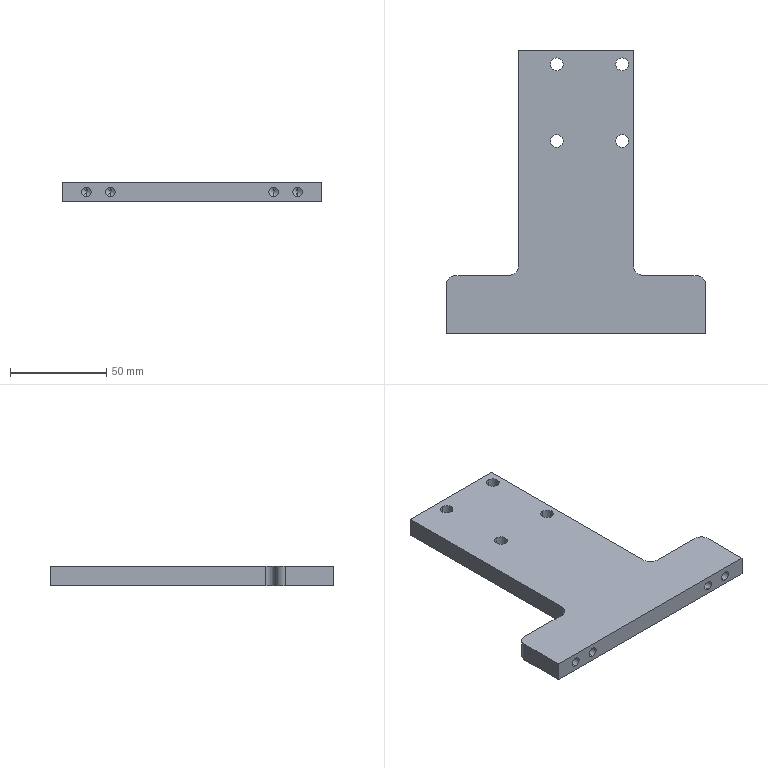Component | SolidWorks | CTM-HVS-52-OA-02-08-01-2 | 1 solid | 46 faces | box 135 x 147 x 10 mm | volume 107309 mm3 | cylinder 24 | cone 12 | plane 10 | commonest cylinder face diameters 5 x12 6.6 x8 10 x4 | material Q235A
build123d program:
from build123d import *

# Parameters (mm, degrees)
EXTRUDE1_DEPTH             = 5
LPATTERN1_COUNT            = 2
LPATTERN1_PITCH            = 40
LPATTERN2_COUNT            = 2
LPATTERN2_PITCH            = 40
M6_TAPPED_HOLE4_AT_2_COUNT = 2
M6_TAPPED_HOLE4_AT_2_PITCH = 12.5
FILLET1_R                  = 5
M6_TAPPED_HOLE2_D          = 5
M6_TAPPED_HOLE2_DEPTH      = 20
M6_TAPPED_HOLE2_TIP        = 1.502
FILLET2_R                  = 5


with BuildPart() as part:
    # Sketch1 → Extrude1 (new, symmetric)
    with BuildSketch(Plane.XY):
        Polygon((-73.5, 30), (-73.5, 67.5), (-43.5, 67.5), (-43.5, 30), (73.5, 30), (73.5, -30), (-43.5, -30), (-43.5, -67.5), (-73.5, -67.5), (-73.5, -30), align=None)
    extrude(amount=EXTRUDE1_DEPTH, both=True)

    # Sketch5 → M6 Clearance Hole1 (revolve, cut)
    with BuildSketch(Plane(origin=(66.5, -10, 5), x_dir=(0, -1, 0), z_dir=(1, 0, 0))):
        Polygon((0, 0), (0, 36.983), (3.3, 35), (3.3, 0), align=None)
    m6_clearance_hole1 = revolve(axis=Axis((66.5, -10, 11.35), (0, 0, -1)), mode=Mode.SUBTRACT)

    # LPattern1: M6 Clearance Hole1 ×2
    with Locations(*[(-i * LPATTERN1_PITCH, 0, 0) for i in range(1, LPATTERN1_COUNT)]):
        add(m6_clearance_hole1, mode=Mode.SUBTRACT)

    # Sketch8 → M6 Clearance Hole2 (revolve, cut)
    with BuildSketch(Plane(origin=(26.5, 24, 5), x_dir=(0, -1, 0), z_dir=(1, 0, 0))):
        Polygon((0, 0), (0, 36.983), (3.3, 35), (3.3, 0), align=None)
    m6_clearance_hole2 = revolve(axis=Axis((26.5, 24, 11.35), (0, 0, -1)), mode=Mode.SUBTRACT)

    # LPattern2: M6 Clearance Hole2 ×2
    with Locations(*[(i * LPATTERN2_PITCH, 0, 0) for i in range(1, LPATTERN2_COUNT)]):
        add(m6_clearance_hole2, mode=Mode.SUBTRACT)

    # Sketch9 → M6 Tapped Hole4 (revolve, cut)
    with BuildSketch(Plane(origin=(-73.5, 42.5, 0), x_dir=(0, 0, 1), z_dir=(0, 1, 0))):
        Polygon((0, 0), (0, 16.502), (2.5, 15), (2.5, 0), align=None)
    m6_tapped_hole4 = revolve(axis=Axis((-79.85, 42.5, 0), (1, 0, 0)), mode=Mode.SUBTRACT)

    # M6 Tapped Hole4 at 2: M6 Tapped Hole4 ×2
    with Locations(*[(0, i * M6_TAPPED_HOLE4_AT_2_PITCH, 0) for i in range(1, M6_TAPPED_HOLE4_AT_2_COUNT)]):
        add(m6_tapped_hole4, mode=Mode.SUBTRACT)

    # Mirror1: M6 Tapped Hole4 across plane
    add(m6_tapped_hole4.mirror(Plane.ZX), mode=Mode.SUBTRACT)

    # Mirror1 copy 1 sketch → Mirror1 copy 1 (revolve, cut)
    with BuildSketch(Plane(origin=(-73.5, -55, 0), x_dir=(0, 0, 1), z_dir=(0, -1, 0))):
        Polygon((0, 0), (0, -16.502), (2.5, -15), (2.5, 0), align=None)
    revolve(axis=Axis((-79.85, -55, 0), (-1, 0, 0)), mode=Mode.SUBTRACT)

    # Mirror2 copy 1 sketch → Mirror2 copy 1 (revolve, cut)
    with BuildSketch(Plane(origin=(-73.5, 42.5, 0), x_dir=(0, 0, 1), z_dir=(0, 1, 0))):
        Polygon((0, 0), (0, 16.502), (2.5, 15), (2.5, 0), align=None)
    revolve(axis=Axis((-79.85, 42.5, 0), (1, 0, 0)), mode=Mode.SUBTRACT)

    # Mirror2 copy 2 sketch → Mirror2 copy 2 (revolve, cut)
    with BuildSketch(Plane(origin=(-73.5, 55, 0), x_dir=(0, 0, 1), z_dir=(0, 1, 0))):
        Polygon((0, 0), (0, 16.502), (2.5, 15), (2.5, 0), align=None)
    revolve(axis=Axis((-79.85, 55, 0), (1, 0, 0)), mode=Mode.SUBTRACT)

    # Mirror2 copy 3 sketch → Mirror2 copy 3 (revolve, cut)
    with BuildSketch(Plane(origin=(-73.5, -42.5, 0), x_dir=(0, 0, 1), z_dir=(0, -1, 0))):
        Polygon((0, 0), (0, -16.502), (2.5, -15), (2.5, 0), align=None)
    revolve(axis=Axis((-79.85, -42.5, 0), (-1, 0, 0)), mode=Mode.SUBTRACT)

    # Mirror2 copy 4 sketch → Mirror2 copy 4 (revolve, cut)
    with BuildSketch(Plane(origin=(-73.5, -55, 0), x_dir=(0, 0, 1), z_dir=(0, -1, 0))):
        Polygon((0, 0), (0, -16.502), (2.5, -15), (2.5, 0), align=None)
    revolve(axis=Axis((-79.85, -55, 0), (-1, 0, 0)), mode=Mode.SUBTRACT)

    # Fillet1
    fillet1_edges = [part.edges().sort_by_distance(p)[0] for p in [
        (-43.5, -30, 0),
        (-43.5, 30, 0),
    ]]
    fillet(fillet1_edges, radius=FILLET1_R)

    # M6 Tapped Hole2
    with Locations(Plane(origin=(73.5, 0, 0), x_dir=(0, 0, -1), z_dir=(1, 0, 0))):
        with Locations((0, 15), (0, -20)):
            Hole(M6_TAPPED_HOLE2_D / 2, depth=M6_TAPPED_HOLE2_DEPTH)
            with Locations((0, 0, -(M6_TAPPED_HOLE2_DEPTH + M6_TAPPED_HOLE2_TIP / 2))):  # 118° drill point
                Cone(0, M6_TAPPED_HOLE2_D / 2, M6_TAPPED_HOLE2_TIP, mode=Mode.SUBTRACT)

    # Fillet2
    fillet2_edges = [part.edges().sort_by_distance(p)[0] for p in [
        (-43.5, -67.5, 0),
        (-43.5, 67.5, 0),
    ]]
    fillet(fillet2_edges, radius=FILLET2_R)


solid = part.part

# Placed as in the assembly
solid = solid.moved(Location((-292.307, 8.943, 385), (180, 0, -90)))